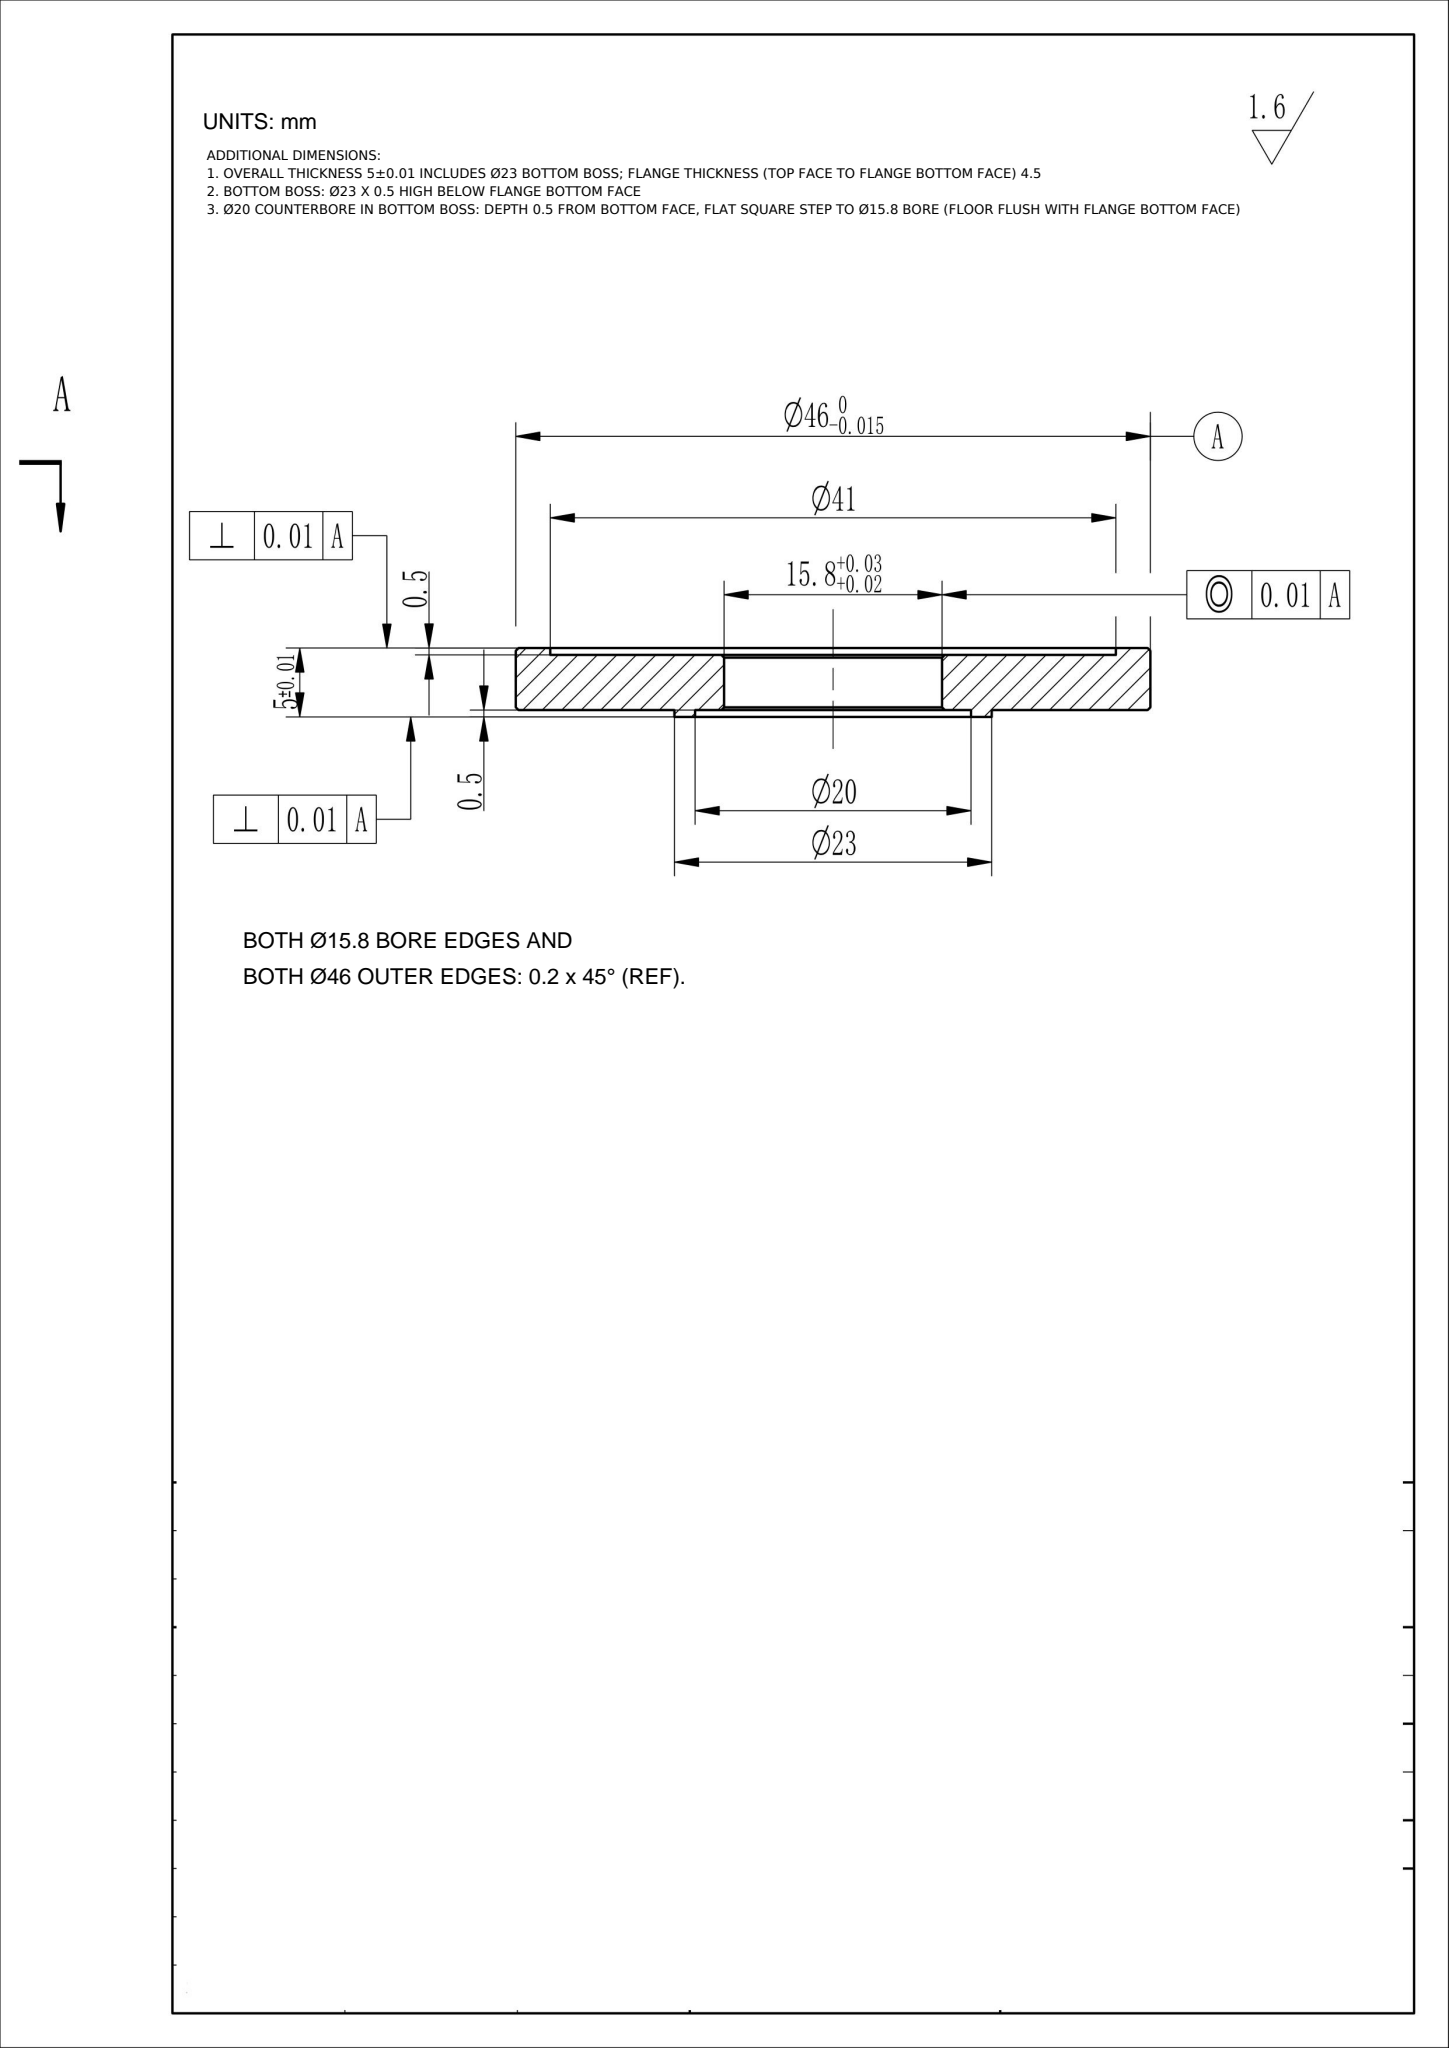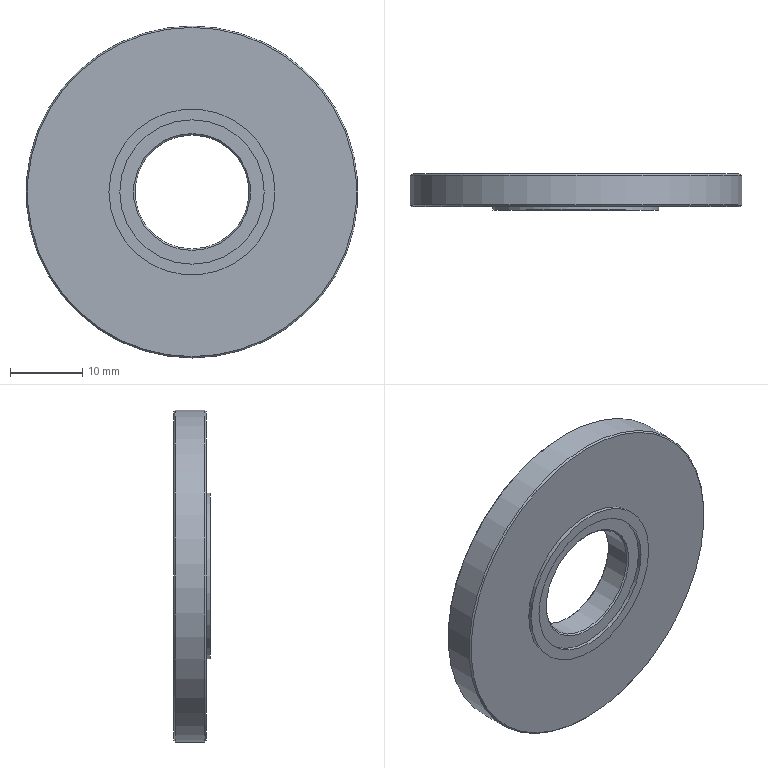Part | NX | mm | 1 solid | 14 faces | box 46 x 5 x 46 mm | volume 6077 mm3 | plane 5 | cylinder 5 | cone 4 | commonest cylinder face diameters 46 x1 15.8 x1 23 x1 20 x1 41 x1
STEP:
#1=CARTESIAN_POINT('',(0.,0.,0.));
#2=DIRECTION('',(0.,0.,1.));
#3=DIRECTION('',(1.,0.,0.));
#4=AXIS2_PLACEMENT_3D('',#1,#2,#3);
#5=(LENGTH_UNIT()NAMED_UNIT(*)SI_UNIT(.MILLI.,.METRE.));
#6=UNCERTAINTY_MEASURE_WITH_UNIT(LENGTH_MEASURE(0.00002),#5,'','');
#7=(NAMED_UNIT(*)PLANE_ANGLE_UNIT()SI_UNIT($,.RADIAN.));
#8=PLANE_ANGLE_MEASURE_WITH_UNIT(PLANE_ANGLE_MEASURE(0.01745),#7);
#9=DIMENSIONAL_EXPONENTS(0.,0.,0.,0.,0.,0.,0.);
#10=(CONVERSION_BASED_UNIT('',#8)NAMED_UNIT(#9)PLANE_ANGLE_UNIT());
#11=(NAMED_UNIT(*)SI_UNIT($,.STERADIAN.)SOLID_ANGLE_UNIT());
#12=(GEOMETRIC_REPRESENTATION_CONTEXT(3)GLOBAL_UNCERTAINTY_ASSIGNED_CONTEXT((#6))GLOBAL_UNIT_ASSIGNED_CONTEXT((#5,#10,#11))REPRESENTATION_CONTEXT('',''));
#13=SHAPE_REPRESENTATION('',(#4),#12);
#14=CARTESIAN_POINT('',(10.,-2.5,-0.));
#15=VERTEX_POINT('',#14);
#16=CARTESIAN_POINT('',(0.,-2.5,0.));
#17=DIRECTION('',(0.,-1.,0.));
#18=DIRECTION('',(1.,0.,-0.));
#19=AXIS2_PLACEMENT_3D('',#16,#17,#18);
#20=CIRCLE('',#19,10.);
#21=EDGE_CURVE('',#15,#15,#20,.T.);
#22=ORIENTED_EDGE('',*,*,#21,.F.);
#23=EDGE_LOOP('',(#22));
#24=FACE_BOUND('',#23,.T.);
#25=CARTESIAN_POINT('',(11.5,-2.5,-0.));
#26=VERTEX_POINT('',#25);
#27=CARTESIAN_POINT('',(0.,-2.5,0.));
#28=DIRECTION('',(0.,-1.,0.));
#29=DIRECTION('',(1.,0.,-0.));
#30=AXIS2_PLACEMENT_3D('',#27,#28,#29);
#31=CIRCLE('',#30,11.5);
#32=EDGE_CURVE('',#26,#26,#31,.T.);
#33=ORIENTED_EDGE('',*,*,#32,.T.);
#34=EDGE_LOOP('',(#33));
#35=FACE_BOUND('',#34,.T.);
#36=CARTESIAN_POINT('',(0.,-2.5,23.));
#37=DIRECTION('',(0.,1.,0.));
#38=DIRECTION('',(0.,0.,1.));
#39=AXIS2_PLACEMENT_3D('',#36,#37,#38);
#40=PLANE('',#39);
#41=ADVANCED_FACE('',(#24,#35),#40,.F.);
#42=CARTESIAN_POINT('',(0.,2.3,-23.));
#43=VERTEX_POINT('',#42);
#44=CARTESIAN_POINT('',(0.,2.3,0.));
#45=DIRECTION('',(0.,-1.,0.));
#46=DIRECTION('',(0.,0.,-1.));
#47=AXIS2_PLACEMENT_3D('',#44,#45,#46);
#48=CIRCLE('',#47,23.);
#49=EDGE_CURVE('',#43,#43,#48,.T.);
#50=ORIENTED_EDGE('',*,*,#49,.T.);
#51=EDGE_LOOP('',(#50));
#52=FACE_BOUND('',#51,.T.);
#53=CARTESIAN_POINT('',(0.,-1.8,-23.));
#54=VERTEX_POINT('',#53);
#55=CARTESIAN_POINT('',(0.,-1.8,0.));
#56=DIRECTION('',(0.,1.,0.));
#57=DIRECTION('',(0.,0.,-1.));
#58=AXIS2_PLACEMENT_3D('',#55,#56,#57);
#59=CIRCLE('',#58,23.);
#60=EDGE_CURVE('',#54,#54,#59,.T.);
#61=ORIENTED_EDGE('',*,*,#60,.T.);
#62=EDGE_LOOP('',(#61));
#63=FACE_BOUND('',#62,.T.);
#64=CARTESIAN_POINT('',(0.,0.,0.));
#65=DIRECTION('',(0.,-1.,0.));
#66=DIRECTION('',(0.,0.,-1.));
#67=AXIS2_PLACEMENT_3D('',#64,#65,#66);
#68=CYLINDRICAL_SURFACE('',#67,23.);
#69=ADVANCED_FACE('',(#52,#63),#68,.T.);
#70=CARTESIAN_POINT('',(0.,-1.8,-7.9));
#71=VERTEX_POINT('',#70);
#72=CARTESIAN_POINT('',(0.,-1.8,0.));
#73=DIRECTION('',(0.,-1.,0.));
#74=DIRECTION('',(0.,0.,-1.));
#75=AXIS2_PLACEMENT_3D('',#72,#73,#74);
#76=CIRCLE('',#75,7.9);
#77=EDGE_CURVE('',#71,#71,#76,.T.);
#78=ORIENTED_EDGE('',*,*,#77,.T.);
#79=EDGE_LOOP('',(#78));
#80=FACE_BOUND('',#79,.T.);
#81=CARTESIAN_POINT('',(0.,1.8,7.9));
#82=VERTEX_POINT('',#81);
#83=CARTESIAN_POINT('',(0.,1.8,0.));
#84=DIRECTION('',(0.,1.,0.));
#85=DIRECTION('',(0.,0.,1.));
#86=AXIS2_PLACEMENT_3D('',#83,#84,#85);
#87=CIRCLE('',#86,7.9);
#88=EDGE_CURVE('',#82,#82,#87,.T.);
#89=ORIENTED_EDGE('',*,*,#88,.T.);
#90=EDGE_LOOP('',(#89));
#91=FACE_BOUND('',#90,.T.);
#92=CARTESIAN_POINT('',(0.,0.,0.));
#93=DIRECTION('',(0.,-1.,0.));
#94=DIRECTION('',(0.,0.,-1.));
#95=AXIS2_PLACEMENT_3D('',#92,#93,#94);
#96=CYLINDRICAL_SURFACE('',#95,7.9);
#97=ADVANCED_FACE('',(#80,#91),#96,.F.);
#98=CARTESIAN_POINT('',(0.,2.5,-22.8));
#99=VERTEX_POINT('',#98);
#100=CARTESIAN_POINT('',(0.,2.5,0.));
#101=DIRECTION('',(0.,1.,0.));
#102=DIRECTION('',(0.,0.,-1.));
#103=AXIS2_PLACEMENT_3D('',#100,#101,#102);
#104=CIRCLE('',#103,22.8);
#105=EDGE_CURVE('',#99,#99,#104,.T.);
#106=ORIENTED_EDGE('',*,*,#105,.T.);
#107=EDGE_LOOP('',(#106));
#108=FACE_BOUND('',#107,.T.);
#109=CARTESIAN_POINT('',(20.5,2.5,0.));
#110=VERTEX_POINT('',#109);
#111=CARTESIAN_POINT('',(0.,2.5,0.));
#112=DIRECTION('',(0.,1.,0.));
#113=DIRECTION('',(1.,0.,0.));
#114=AXIS2_PLACEMENT_3D('',#111,#112,#113);
#115=CIRCLE('',#114,20.5);
#116=EDGE_CURVE('',#110,#110,#115,.T.);
#117=ORIENTED_EDGE('',*,*,#116,.F.);
#118=EDGE_LOOP('',(#117));
#119=FACE_BOUND('',#118,.T.);
#120=CARTESIAN_POINT('',(0.,2.5,7.9));
#121=DIRECTION('',(0.,-1.,0.));
#122=DIRECTION('',(0.,0.,-1.));
#123=AXIS2_PLACEMENT_3D('',#120,#121,#122);
#124=PLANE('',#123);
#125=ADVANCED_FACE('',(#108,#119),#124,.F.);
#126=CARTESIAN_POINT('',(11.5,-2.,-0.));
#127=VERTEX_POINT('',#126);
#128=CARTESIAN_POINT('',(0.,-2.,0.));
#129=DIRECTION('',(0.,1.,0.));
#130=DIRECTION('',(1.,0.,-0.));
#131=AXIS2_PLACEMENT_3D('',#128,#129,#130);
#132=CIRCLE('',#131,11.5);
#133=EDGE_CURVE('',#127,#127,#132,.T.);
#134=ORIENTED_EDGE('',*,*,#133,.F.);
#135=EDGE_LOOP('',(#134));
#136=FACE_BOUND('',#135,.T.);
#137=ORIENTED_EDGE('',*,*,#32,.F.);
#138=EDGE_LOOP('',(#137));
#139=FACE_BOUND('',#138,.T.);
#140=CARTESIAN_POINT('',(0.,-2.,0.));
#141=DIRECTION('',(0.,-1.,0.));
#142=DIRECTION('',(0.,0.,-1.));
#143=AXIS2_PLACEMENT_3D('',#140,#141,#142);
#144=CYLINDRICAL_SURFACE('',#143,11.5);
#145=ADVANCED_FACE('',(#136,#139),#144,.T.);
#146=CARTESIAN_POINT('',(0.,-2.,-22.8));
#147=VERTEX_POINT('',#146);
#148=CARTESIAN_POINT('',(0.,-2.,0.));
#149=DIRECTION('',(0.,-1.,0.));
#150=DIRECTION('',(0.,0.,-1.));
#151=AXIS2_PLACEMENT_3D('',#148,#149,#150);
#152=CIRCLE('',#151,22.8);
#153=EDGE_CURVE('',#147,#147,#152,.T.);
#154=ORIENTED_EDGE('',*,*,#153,.T.);
#155=EDGE_LOOP('',(#154));
#156=FACE_BOUND('',#155,.T.);
#157=ORIENTED_EDGE('',*,*,#133,.T.);
#158=EDGE_LOOP('',(#157));
#159=FACE_BOUND('',#158,.T.);
#160=CARTESIAN_POINT('',(0.,-2.,0.));
#161=DIRECTION('',(0.,-1.,0.));
#162=DIRECTION('',(0.,0.,-1.));
#163=AXIS2_PLACEMENT_3D('',#160,#161,#162);
#164=PLANE('',#163);
#165=ADVANCED_FACE('',(#156,#159),#164,.T.);
#166=CARTESIAN_POINT('',(10.,-2.,-0.));
#167=VERTEX_POINT('',#166);
#168=CARTESIAN_POINT('',(0.,-2.,0.));
#169=DIRECTION('',(0.,1.,0.));
#170=DIRECTION('',(1.,0.,-0.));
#171=AXIS2_PLACEMENT_3D('',#168,#169,#170);
#172=CIRCLE('',#171,10.);
#173=EDGE_CURVE('',#167,#167,#172,.T.);
#174=ORIENTED_EDGE('',*,*,#173,.T.);
#175=EDGE_LOOP('',(#174));
#176=FACE_BOUND('',#175,.T.);
#177=ORIENTED_EDGE('',*,*,#21,.T.);
#178=EDGE_LOOP('',(#177));
#179=FACE_BOUND('',#178,.T.);
#180=CARTESIAN_POINT('',(0.,-2.,0.));
#181=DIRECTION('',(0.,-1.,0.));
#182=DIRECTION('',(0.,0.,-1.));
#183=AXIS2_PLACEMENT_3D('',#180,#181,#182);
#184=CYLINDRICAL_SURFACE('',#183,10.);
#185=ADVANCED_FACE('',(#176,#179),#184,.F.);
#186=CARTESIAN_POINT('',(0.,-2.,-8.1));
#187=VERTEX_POINT('',#186);
#188=CARTESIAN_POINT('',(0.,-2.,0.));
#189=DIRECTION('',(0.,1.,0.));
#190=DIRECTION('',(0.,0.,-1.));
#191=AXIS2_PLACEMENT_3D('',#188,#189,#190);
#192=CIRCLE('',#191,8.1);
#193=EDGE_CURVE('',#187,#187,#192,.T.);
#194=ORIENTED_EDGE('',*,*,#193,.T.);
#195=EDGE_LOOP('',(#194));
#196=FACE_BOUND('',#195,.T.);
#197=ORIENTED_EDGE('',*,*,#173,.F.);
#198=EDGE_LOOP('',(#197));
#199=FACE_BOUND('',#198,.T.);
#200=CARTESIAN_POINT('',(0.,-2.,0.));
#201=DIRECTION('',(0.,-1.,0.));
#202=DIRECTION('',(0.,0.,-1.));
#203=AXIS2_PLACEMENT_3D('',#200,#201,#202);
#204=PLANE('',#203);
#205=ADVANCED_FACE('',(#196,#199),#204,.T.);
#206=CARTESIAN_POINT('',(20.5,2.,0.));
#207=VERTEX_POINT('',#206);
#208=CARTESIAN_POINT('',(0.,2.,0.));
#209=DIRECTION('',(0.,-1.,0.));
#210=DIRECTION('',(1.,0.,0.));
#211=AXIS2_PLACEMENT_3D('',#208,#209,#210);
#212=CIRCLE('',#211,20.5);
#213=EDGE_CURVE('',#207,#207,#212,.T.);
#214=ORIENTED_EDGE('',*,*,#213,.T.);
#215=EDGE_LOOP('',(#214));
#216=FACE_BOUND('',#215,.T.);
#217=ORIENTED_EDGE('',*,*,#116,.T.);
#218=EDGE_LOOP('',(#217));
#219=FACE_BOUND('',#218,.T.);
#220=CARTESIAN_POINT('',(0.,2.,0.));
#221=DIRECTION('',(0.,1.,0.));
#222=DIRECTION('',(0.,0.,1.));
#223=AXIS2_PLACEMENT_3D('',#220,#221,#222);
#224=CYLINDRICAL_SURFACE('',#223,20.5);
#225=ADVANCED_FACE('',(#216,#219),#224,.F.);
#226=CARTESIAN_POINT('',(0.,2.,8.1));
#227=VERTEX_POINT('',#226);
#228=CARTESIAN_POINT('',(0.,2.,0.));
#229=DIRECTION('',(0.,-1.,0.));
#230=DIRECTION('',(0.,0.,1.));
#231=AXIS2_PLACEMENT_3D('',#228,#229,#230);
#232=CIRCLE('',#231,8.1);
#233=EDGE_CURVE('',#227,#227,#232,.T.);
#234=ORIENTED_EDGE('',*,*,#233,.T.);
#235=EDGE_LOOP('',(#234));
#236=FACE_BOUND('',#235,.T.);
#237=ORIENTED_EDGE('',*,*,#213,.F.);
#238=EDGE_LOOP('',(#237));
#239=FACE_BOUND('',#238,.T.);
#240=CARTESIAN_POINT('',(0.,2.,0.));
#241=DIRECTION('',(0.,1.,0.));
#242=DIRECTION('',(0.,0.,1.));
#243=AXIS2_PLACEMENT_3D('',#240,#241,#242);
#244=PLANE('',#243);
#245=ADVANCED_FACE('',(#236,#239),#244,.T.);
#246=ORIENTED_EDGE('',*,*,#193,.F.);
#247=EDGE_LOOP('',(#246));
#248=FACE_BOUND('',#247,.T.);
#249=ORIENTED_EDGE('',*,*,#77,.F.);
#250=EDGE_LOOP('',(#249));
#251=FACE_BOUND('',#250,.T.);
#252=CARTESIAN_POINT('',(0.,-1.8,0.));
#253=DIRECTION('',(0.,-1.,0.));
#254=DIRECTION('',(0.,-0.,-1.));
#255=AXIS2_PLACEMENT_3D('',#252,#253,#254);
#256=CONICAL_SURFACE('',#255,7.9,45.);
#257=ADVANCED_FACE('',(#248,#251),#256,.F.);
#258=ORIENTED_EDGE('',*,*,#233,.F.);
#259=EDGE_LOOP('',(#258));
#260=FACE_BOUND('',#259,.T.);
#261=ORIENTED_EDGE('',*,*,#88,.F.);
#262=EDGE_LOOP('',(#261));
#263=FACE_BOUND('',#262,.T.);
#264=CARTESIAN_POINT('',(0.,1.8,0.));
#265=DIRECTION('',(0.,1.,0.));
#266=DIRECTION('',(0.,0.,1.));
#267=AXIS2_PLACEMENT_3D('',#264,#265,#266);
#268=CONICAL_SURFACE('',#267,7.9,45.);
#269=ADVANCED_FACE('',(#260,#263),#268,.F.);
#270=ORIENTED_EDGE('',*,*,#105,.F.);
#271=EDGE_LOOP('',(#270));
#272=FACE_BOUND('',#271,.T.);
#273=ORIENTED_EDGE('',*,*,#49,.F.);
#274=EDGE_LOOP('',(#273));
#275=FACE_BOUND('',#274,.T.);
#276=CARTESIAN_POINT('',(0.,2.3,0.));
#277=DIRECTION('',(0.,-1.,0.));
#278=DIRECTION('',(0.,-0.,-1.));
#279=AXIS2_PLACEMENT_3D('',#276,#277,#278);
#280=CONICAL_SURFACE('',#279,23.,45.);
#281=ADVANCED_FACE('',(#272,#275),#280,.T.);
#282=ORIENTED_EDGE('',*,*,#60,.F.);
#283=EDGE_LOOP('',(#282));
#284=FACE_BOUND('',#283,.T.);
#285=ORIENTED_EDGE('',*,*,#153,.F.);
#286=EDGE_LOOP('',(#285));
#287=FACE_BOUND('',#286,.T.);
#288=CARTESIAN_POINT('',(0.,-2.,0.));
#289=DIRECTION('',(0.,1.,0.));
#290=DIRECTION('',(0.,-0.,1.));
#291=AXIS2_PLACEMENT_3D('',#288,#289,#290);
#292=CONICAL_SURFACE('',#291,22.8,45.);
#293=ADVANCED_FACE('',(#284,#287),#292,.T.);
#294=CLOSED_SHELL('',(#41,#69,#97,#125,#145,#165,#185,#205,#225,#245,#257,#269,#281,#293));
#295=MANIFOLD_SOLID_BREP('',#294);
#296=ADVANCED_BREP_SHAPE_REPRESENTATION('',(#295),#12);
#297=SHAPE_REPRESENTATION_RELATIONSHIP('','',#13,#296);
#298=PRESENTATION_LAYER_ASSIGNMENT('','',(#295));
#299=COLOUR_RGB('',1.,0.6,0.);
#300=FILL_AREA_STYLE_COLOUR('',#299);
#301=FILL_AREA_STYLE('',(#300));
#302=SURFACE_STYLE_FILL_AREA(#301);
#303=SURFACE_SIDE_STYLE('',(#302));
#304=SURFACE_STYLE_USAGE(.BOTH.,#303);
#305=PRESENTATION_STYLE_ASSIGNMENT((#304));
#306=STYLED_ITEM('',(#305),#295);
#307=MECHANICAL_DESIGN_GEOMETRIC_PRESENTATION_REPRESENTATION('',(#306),#12);